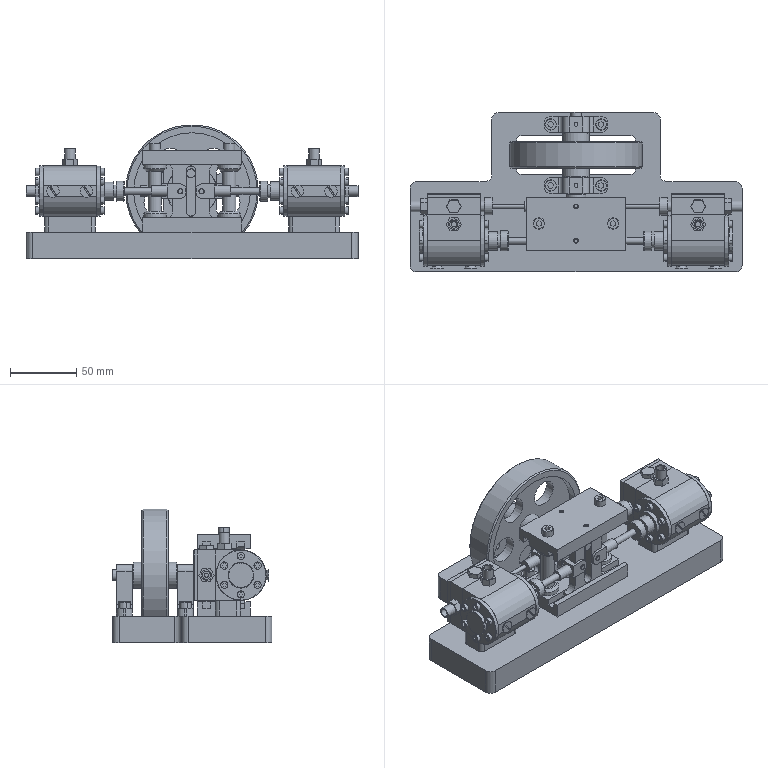Assembly | NX | mm | 90 component files | 90 solids | 1721 faces | box 250 x 120.25 x 101 mm | volume 767415 mm3 | plane 811 | cylinder 535 | cone 233 | torus 142 | commonest cylinder face diameters 3 x80 5 x80 4 x76 5.5 x48 8 x47 10 x32 4.2 x24 19 x16
Bill of materials:
unnamed part 1 | 2 |  | Short cylindrical disk with a rectangular circumferential groove between two equal flanges and a central axial through hole; one end face appears to have a larger shallow recess around the hole.
unnamed part 2 | 1 |  | Wheel-like disk with five equally spaced round lightening holes, a central cylindrical hub boss sticking out from both faces with a small axial bore, a slightly recessed face inside an outer rim, and chamfered outer edges.
unnamed part 3 | 2 |  | Thin flat rectangular plate with eight round through holes near the edges, two on each side.
unnamed part 4 | 4 |  | Fastener-like solid with a conical countersunk-style flat head, a straight slot across the head face, a filleted reduced-diameter neck, and a larger plain cylindrical shank with a chamfered end.
unnamed part 5 | 2 |  | Rectangular block frame with a large rectangular through window, eight round holes through the main face around the window, large round cross holes through the top/bottom and side walls, and a small hole in one side wall.
unnamed part 6 | 1 |  | Flat plate with a T-shaped outline: a wide rectangular base with a narrower rectangular tab, rounded outer corners and filleted inside corners. The tab has a rounded-rectangle cutout and four holes, and the base has two holes and two clusters of six small holes.
unnamed part 7 | 4 |  | Hollow straight-through body with a central hexagonal collar and equal cylindrical tube sections on both sides, all sharing one round through bore.
unnamed part 8 | 2 |  | Circular flange disk with six equally spaced bolt-circle holes and a central through hole. A cylindrical hub stands out from one face, and a larger-diameter short boss stands out slightly from the opposite face.
unnamed part 9 | 1 |  | Thick flat plate with an I-shaped outline: large concave arcs cut into both long sides, a long central slot with round ends, and two shorter round-ended slots on either side of it.
unnamed part 10 | 2 |  | Solid body with a hexagonal head, chamfered top edges, and a plain cylindrical shank with a chamfered end.
unnamed part 11 | 24 |  | Fastener-like body with a plain cylindrical head and a long smaller-diameter plain cylindrical shank with a chamfered tip.
unnamed part 12 | 2 |  | Block with one long side rounded to a half-cylinder, a large axial through bore with a small keyway notch, six holes with conical bottoms on a circle on the end face, a small through hole next to the bore, two holes on a side face and one hole on the top face.
unnamed part 13 | 1 |  | Thin circular disc with a long slender cylindrical rod projecting from the center of one face and a short, smaller cylindrical pin projecting off-center from the opposite face.
unnamed part 14 | 2 |  | Rectangular plate with a narrower rectangular block on one face; the block has a round through hole crossing it parallel to the plate. The large face appears to have a shallow stepped or recessed border region.
unnamed part 15 | 2 |  | Rectangular block with rounded vertical corners, pierced by six through holes: two larger holes on the long centerline and four smaller holes near the corners.
unnamed part 16 | 2 |  | Upright bracket with a flat base having rounded ends and two through holes, and a central vertical web with a rounded top containing a large horizontal through hole; a small hole enters the top face of the upright.
unnamed part 17 | 2 |  | Clevis-like part: rectangular block with an open slot forming two parallel prongs with rounded ends, a cross hole through both prongs, and a cylindrical shank with an axial bore extending from the opposite side.
unnamed part 18 | 2 |  | Socket-head-screw-shaped part: cylindrical head with hexagonal recess on top and a smooth cylindrical shank with a chamfered tip.
unnamed part 19 | 1 |  | Flat plate with constant thickness and an H-like outline formed by large rounded notches on two opposite sides, a central obround through opening, and two small obround slots on either side of it.
unnamed part 20 | 2 |  | Long solid cylindrical pin with a single step to a shorter, reduced-diameter section at one end.
unnamed part 21 | 2 |  | Rectangular frame block with a large square through opening and a round through hole crossing the two side walls on a shared axis.
unnamed part 22 | 2 |  | Plain long slender solid cylindrical rod with flat ends.
unnamed part 23 | 1 |  | Flanged bushing-like cylinder: a larger-diameter flange and a smaller-diameter cylindrical body, with a round through bore and small edge chamfers.
unnamed part 24 | 2 |  | Clevis-like part like the other forked part: slotted rectangular block with two rounded-end prongs and a cross hole, plus a cylindrical shank; here the shank has a smaller axial hole that appears to end in a conical bottom.
unnamed part 25 | 2 |  | Flat circular disc with six evenly spaced round through holes on a bolt circle and a smaller raised circular boss in the middle. The center is solid.
unnamed part 26 | 2 |  | Stepped solid of revolution: a larger-diameter cylinder joined to a smaller-diameter cylinder, with a small hole along the central axis. Outer edges are chamfered.
unnamed part 27 | 2 |  | Rectangular block with four through holes in the top face (two larger and two smaller) and two parallel rectangular grooves cut into the underside.
unnamed part 28 | 4 |  | Screw-like part: a cylindrical head with a hexagonal socket recess on top a plain cylindrical shank with a chamfered tip. It resembles a socket head cap screw.
unnamed part 29 | 2 |  | Flat split ring with a rectangular cross-section and one narrow gap through its circumference.
unnamed part 30 | 2 |  | Spool-shaped solid of revolution: a central cylindrical shaft between two larger flat end flanges, with a chamfered transition where each flange meets the shaft. There is a central hole at the end.
unnamed part 31 | 4 |  | Solid cylinder (pin shape) with chamfered edges at both ends.
unnamed part 32 | 2 |  | Flanged bushing shape: a larger cylindrical collar joined to a smaller tubular section, with a central bore through both.
unnamed part 33 | 2 |  | Pin or screw-like part: a long plain cylindrical shank with a chamfered tip and a short cylindrical head of larger diameter at the other end.
Mates:
1. fix | Base_Plate 1 component
2. concentric | Piston_Cylinder_Link_Platform 2 arc | Base_Plate 1 edge
3. parallel | Piston_Cylinder_Link_Platform 2 face | Base_Plate 1 face
4. concentric | Base_Plate 1 edge | Piston_Cylinder_Link_Platform 1 arc
5. parallel | Piston_Cylinder_Link_Platform 1 face | Base_Plate 1 face
6. concentric | Base_Plate 1 edge | Middle_Support_Platform 2 edge
7. parallel | Middle_Support_Platform 2 face | Base_Plate 1 face
8. touch align | Piston_Cylinder 2 face | Piston_Cylinder_Link_Platform 1 face
9. center | Piston_Cylinder 2 face | Piston_Cylinder 2 face | Piston_Cylinder_Link_Platform 1 face | Piston_Cylinder_Link_Platform 1 face
10. touch align | Piston_Cylinder 1 face | Piston_Cylinder_Link_Platform 2 face
11. center | Piston_Cylinder 1 face | Piston_Cylinder 1 face | Piston_Cylinder_Link_Platform 2 face | Piston_Cylinder_Link_Platform 2 face
12. touch align | Piston_Cylinder 1 face | Piston_Cylinder_Link_Platform 2 face
13. touch align | Piston_Cylinder 1 face | Piston_Cylinder 2 face
14. concentric | Middle_Support_Platform 2 edge | Pillar 2 edge
15. concentric | Pillar 1 edge | Middle_Support_Platform 2 edge
16. concentric | Middle_Support_Platform 1 arc | Pillar 2 edge
17. parallel | Middle_Support_Platform 1 face | Middle_Support_Platform 2 face
18. concentric | Support_Seat 2 edge | Base_Plate 1 edge
19. parallel | Support_Seat 2 face | Base_Plate 1 face
20. concentric | Support_Seat 1 edge | Base_Plate 1 edge
21. parallel | Support_Seat 1 face | Support_Seat 2 face
22. center | Middle_Support_Platform 2 face | Middle_Support_Platform 2 face | Piston_Cylinder 2 face
23. concentric | External_Piston_Cylinder_Body 2 edge | Piston_Cylinder 2 edge
24. parallel | External_Piston_Cylinder_Body 2 face | Piston_Cylinder 2 face
25. concentric | External_Piston_Cylinder_Body 1 edge | Piston_Cylinder 1 edge
26. parallel | External_Piston_Cylinder_Body 1 face | Piston_Cylinder 1 face
27. touch align | Slide_Plate_1 1 face | Middle_Support_Platform 2 face
28. center | Slide_Plate_1 1 face | Slide_Plate_1 1 face | Middle_Support_Platform 2 face | Middle_Support_Platform 2 face
29. touch align | Middle_Support_Platform 2 face | Slide_Plate_2 1 face
30. center | Slide_Plate_2 1 face | Slide_Plate_2 1 face | Middle_Support_Platform 2 face | Middle_Support_Platform 2 face
31. touch align | Flywheel 1 face | Support_Seat 1 face
32. center | Flywheel 1 face | Flywheel 1 face | Support_Seat 1 face | Support_Seat 2 face
33. center | Connecting_Rod_Joint_1 2 face | Connecting_Rod_Joint_1 2 face | Slide_Plate_1 1 face | Slide_Plate_1 1 face
34. center | Slide_Plate_1 1 face | Slide_Plate_1 1 face | Connecting_Rod_Joint_1 2 face
35. concentric | Piston_Rod_1 2 edge | Connecting_Rod_Joint_1 2 edge
36. concentric | Piston_Rod_1 2 edge | Piston 2 edge
37. concentric | Piston_Ring 2 arc | Piston 2 edge
38. touch align | Connecting_Rod_Joint_1_Connecting_Shaft 4 face | Connecting_Rod_Joint_1 2 face
39. center | Connecting_Rod_Joint_1_Connecting_Shaft 4 face | Connecting_Rod_Joint_1_Connecting_Shaft 4 face | Connecting_Rod_Joint_1 2 face | Connecting_Rod_Joint_1 2 face
40. center | Connecting_Rod_Joint_1 1 face | Connecting_Rod_Joint_1 1 face | Slide_Plate_1 1 face | Slide_Plate_1 1 face
41. center | Slide_Plate_1 1 face | Slide_Plate_1 1 face | Connecting_Rod_Joint_1 1 face
42. center | Slide_Plate_1 1 face | Slide_Plate_1 1 face | Connecting_Rod_Joint_1 1 face
43. concentric | Piston_Rod_1 1 edge | Connecting_Rod_Joint_1 1 edge
44. concentric | Piston_Rod_1 1 edge | Piston 1 edge
45. concentric | Piston_Ring 1 arc | Piston 1 edge
46. touch align | Piston_Rod_1 2 face | Piston_Cylinder 2 face
47. touch align | Piston_Rod_1 1 face | Piston_Cylinder 1 face
48. touch align | Connecting_Rod_Joint_1_Connecting_Shaft 3 face | Connecting_Rod_Joint_1 1 face
49. center | Connecting_Rod_Joint_1_Connecting_Shaft 3 face | Connecting_Rod_Joint_1_Connecting_Shaft 3 face | Connecting_Rod_Joint_1 1 face | Connecting_Rod_Joint_1 1 face
50. touch align | Crankshaft 1 face | Support_Seat 2 face
51. center | Slide_Plate_1 1 face | Slide_Plate_1 1 face | Crankshaft 1 face
52. touch align | Eccentric_Wheel 1 face | Crankshaft 1 face
53. touch align | Crankshaft 1 face | Slide_Plate_1 1 face
54. touch align | Eccentric_Wheel 1 face | Slide_Plate_2 1 face
55. touch align | Eccentric_Wheel 1 face | Slide_Plate_2 1 face
56. bond | Flywheel 1 component | Crankshaft 1 component
57. concentric | External_Piston_Cylinder_Head 2 arc | External_Piston_Cylinder_Body 1 edge
58. parallel | External_Piston_Cylinder_Head 2 face | External_Piston_Cylinder_Body 1 face
59. concentric | External_Piston_Cylinder_Head 1 arc | External_Piston_Cylinder_Body 2 edge
60. parallel | External_Piston_Cylinder_Head 1 face | External_Piston_Cylinder_Body 2 face
61. center | Connecting_Rod_Joint_2 2 face | Connecting_Rod_Joint_2 2 face | Slide_Plate_2 1 face | Slide_Plate_2 1 face
62. center | Slide_Plate_2 1 face | Slide_Plate_2 1 face | Connecting_Rod_Joint_2 2 face
63. concentric | Piston_Rod_2 2 edge | Connecting_Rod_Joint_2 2 edge
64. touch align | Piston_Rod_2 2 face | External_Piston_Cylinder_Body 2 face
65. center | Connecting_Rod_Joint_2 1 face | Connecting_Rod_Joint_2 1 face | Slide_Plate_2 1 face | Slide_Plate_2 1 face
66. touch align | Piston_Rod_2 1 face | External_Piston_Cylinder_Body 1 face
67. concentric | Piston_Rod_2 1 edge | Connecting_Rod_Joint_2 1 edge
68. touch align | Outer_Piston_Block 2 face | Piston_Rod_2 1 face
69. parallel | Outer_Piston_Block 2 face | External_Piston_Cylinder_Body 1 face
70. touch align | Piston_Block_Assembly 2 face | Piston_Rod_2 1 face
71. parallel | Piston_Block_Assembly 2 face | External_Piston_Cylinder_Body 1 face
72. center | Piston_Block_Assembly 2 face | Piston_Block_Assembly 2 face | Outer_Piston_Block 2 face | Outer_Piston_Block 2 face
73. touch align | Piston_Rod_2 1 face | Piston_Block_Assembly 2 face
74. touch align | Outer_Piston_Block 1 face | Piston_Rod_2 2 face
75. parallel | Outer_Piston_Block 1 face | External_Piston_Cylinder_Body 2 face
76. touch align | Piston_Block_Assembly 1 face | Piston_Rod_2 2 face
77. center | Piston_Block_Assembly 1 face | Piston_Block_Assembly 1 face | Outer_Piston_Block 1 face | Outer_Piston_Block 1 face
78. parallel | Piston_Block_Assembly 1 face | External_Piston_Cylinder_Body 2 face
79. touch align | Piston_Rod_2 2 face | Piston_Block_Assembly 1 face
80. touch align | Connecting_Rod_Joint_1_Connecting_Shaft 2 face | Connecting_Rod_Joint_2 2 face
81. center | Connecting_Rod_Joint_1_Connecting_Shaft 2 face | Connecting_Rod_Joint_1_Connecting_Shaft 2 face | Connecting_Rod_Joint_2 2 face | Connecting_Rod_Joint_2 2 face
82. touch align | Connecting_Rod_Joint_1_Connecting_Shaft 1 face | Connecting_Rod_Joint_2 1 face
83. center | Connecting_Rod_Joint_1_Connecting_Shaft 1 face | Connecting_Rod_Joint_1_Connecting_Shaft 1 face | Connecting_Rod_Joint_2 1 face | Connecting_Rod_Joint_2 1 face
84. center | Slide_Plate_2 1 face | Slide_Plate_2 1 face | Connecting_Rod_Joint_1_Connecting_Shaft 1 face
85. concentric | Piston_Cylinder 2 edge | Outer_End_Cover 2 edge
86. concentric | Outer_End_Cover 2 edge | Piston_Cylinder 2 edge
87. concentric | Outer_End_Cover 1 edge | Piston_Cylinder 1 edge
88. concentric | Outer_End_Cover 1 edge | Piston_Cylinder 1 edge
89. concentric | Hex_Socket_Cap_Screw_M3x10 24 edge | Outer_End_Cover 2 edge
90. bond | Outer_End_Cover 2 component | assembly component
91. bond | Hex_Socket_Cap_Screw_M3x10 24 component | assembly component
92. bond | Hex_Socket_Cap_Screw_M3x10 23 component | assembly component
93. bond | Hex_Socket_Cap_Screw_M3x10 22 component | assembly component
94. circular | assembly datumaxis | assembly cartesiancoordinatesystem | assembly cartesiancoordinatesystem | assembly cartesiancoordinatesystem | assembly cartesiancoordinatesystem | assembly cartesiancoordinatesystem | assembly cartesiancoordinatesystem
95. bond | Hex_Socket_Cap_Screw_M3x10 21 component | assembly component
96. bond | Hex_Socket_Cap_Screw_M3x10 20 component | assembly component
97. bond | Hex_Socket_Cap_Screw_M3x10 19 component | assembly component
98. concentric | Hex_Socket_Cap_Screw_M3x10 18 edge | Outer_End_Cover 1 edge
99. bond | Outer_End_Cover 1 component | assembly component
100. bond | Hex_Socket_Cap_Screw_M3x10 18 component | assembly component
101. bond | Hex_Socket_Cap_Screw_M3x10 17 component | assembly component
102. bond | Hex_Socket_Cap_Screw_M3x10 16 component | assembly component
103. bond | Hex_Socket_Cap_Screw_M3x10 15 component | assembly component
104. bond | Hex_Socket_Cap_Screw_M3x10 14 component | assembly component
105. bond | Hex_Socket_Cap_Screw_M3x10 13 component | assembly component
106. circular | assembly datumaxis | assembly cartesiancoordinatesystem | assembly cartesiancoordinatesystem | assembly cartesiancoordinatesystem | assembly cartesiancoordinatesystem | assembly cartesiancoordinatesystem | assembly cartesiancoordinatesystem
107. concentric | Front_End_Cover 2 edge | Piston_Cylinder 2 edge
108. touch align | Front_End_Cover 2 face | Piston_Cylinder 2 face
109. concentric | Front_End_Cover 1 edge | Piston_Cylinder 1 edge
110. concentric | Front_End_Cover 1 edge | Piston_Cylinder 1 edge
111. concentric | Port_1 2 edge | Front_End_Cover 2 edge
112. concentric | Port_1 1 edge | Front_End_Cover 1 edge
113. concentric | Port_2 2 edge | External_Piston_Cylinder_Body 1 edge
114. concentric | Port_2 1 edge | External_Piston_Cylinder_Body 2 edge
115. concentric | External_Piston_Cylinder_Body 2 edge | Bolt 2 edge
116. concentric | External_Piston_Cylinder_Body 1 edge | Bolt 1 edge
117. concentric | Hex_Socket_Cap_Screw_M3x10 12 edge | Front_End_Cover 2 edge
118. bond | Front_End_Cover 2 component | assembly component
119. bond | Hex_Socket_Cap_Screw_M3x10 12 component | assembly component
120. bond | Hex_Socket_Cap_Screw_M3x10 11 component | assembly component
121. bond | Hex_Socket_Cap_Screw_M3x10 10 component | assembly component
122. bond | Hex_Socket_Cap_Screw_M3x10 9 component | assembly component
123. bond | Hex_Socket_Cap_Screw_M3x10 8 component | assembly component
124. bond | Hex_Socket_Cap_Screw_M3x10 7 component | assembly component
125. circular | assembly datumaxis | assembly cartesiancoordinatesystem | assembly cartesiancoordinatesystem | assembly cartesiancoordinatesystem | assembly cartesiancoordinatesystem | assembly cartesiancoordinatesystem | assembly cartesiancoordinatesystem
126. concentric | Hex_Socket_Cap_Screw_M3x10 6 edge | Front_End_Cover 1 edge
127. bond | Front_End_Cover 1 component | assembly component
128. bond | Hex_Socket_Cap_Screw_M3x10 6 component | assembly component
129. bond | Hex_Socket_Cap_Screw_M3x10 5 component | assembly component
130. bond | Hex_Socket_Cap_Screw_M3x10 4 component | assembly component
131. bond | Hex_Socket_Cap_Screw_M3x10 3 component | assembly component
132. bond | Hex_Socket_Cap_Screw_M3x10 2 component | assembly component
133. bond | Hex_Socket_Cap_Screw_M3x10 1 component | assembly component
134. circular | assembly datumaxis | assembly cartesiancoordinatesystem | assembly cartesiancoordinatesystem | assembly cartesiancoordinatesystem | assembly cartesiancoordinatesystem | assembly cartesiancoordinatesystem | assembly cartesiancoordinatesystem
135. concentric | Piston_Cylinder 2 edge | Pipe_Cap_Interface 4 edge
136. parallel | Pipe_Cap_Interface 4 face | Base_Plate 1 face
137. concentric | Piston_Cylinder 1 edge | Pipe_Cap_Interface 3 edge
138. parallel | Pipe_Cap_Interface 3 face | Base_Plate 1 face
139. concentric | Pipe_Cap_Interface 2 edge | External_Piston_Cylinder_Body 2 edge
140. parallel | Pipe_Cap_Interface 2 face | External_Piston_Cylinder_Body 2 face
141. concentric | External_Piston_Cylinder_Body 1 edge | Pipe_Cap_Interface 1 edge
142. parallel | Pipe_Cap_Interface 1 face | External_Piston_Cylinder_Body 1 face
143. touch align | Slotted_Countersunk_Screw_M5x10 4 face | Piston_Cylinder 2 face
144. touch align | Piston_Cylinder 2 face | Slotted_Countersunk_Screw_M5x10 4 face
145. touch align | Slotted_Countersunk_Screw_M5x10 3 face | Piston_Cylinder 2 face
146. touch align | Piston_Cylinder 2 face | Slotted_Countersunk_Screw_M5x10 3 face
147. touch align | Slotted_Countersunk_Screw_M5x10 2 face | Piston_Cylinder 1 face
148. touch align | Piston_Cylinder 1 face | Slotted_Countersunk_Screw_M5x10 2 face
149. touch align | Slotted_Countersunk_Screw_M5x10 1 face | Piston_Cylinder 1 face
150. touch align | Piston_Cylinder 1 face | Slotted_Countersunk_Screw_M5x10 1 face
151. concentric | Hex_Socket_Cap_Screw_M5x16 2 edge | Middle_Support_Platform 1 edge
152. concentric | Hex_Socket_Cap_Screw_M5x16 1 edge | Middle_Support_Platform 1 edge
153. concentric | Hex_Socket_Cap_Screw_M5x25 4 edge | Support_Seat 1 edge
154. concentric | Hex_Socket_Cap_Screw_M5x25 3 edge | Support_Seat 2 edge
155. concentric | Hex_Socket_Cap_Screw_M5x25 2 edge | Support_Seat 2 edge
156. concentric | Hex_Socket_Cap_Screw_M5x25 1 edge | Support_Seat 1 edge
157. concentric | Hex_Socket_Cap_Screw_M5x30 2 edge | Base_Plate 1 edge
158. concentric | Hex_Socket_Cap_Screw_M5x30 1 edge | Base_Plate 1 edge